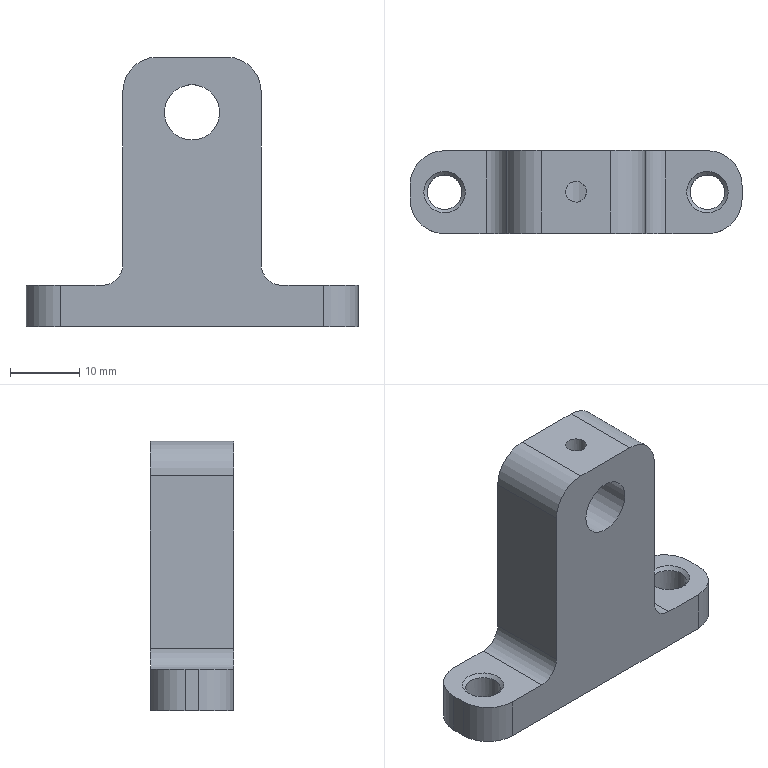Component | NX | SUPPORT_SEAT_2 | 1 solid | 24 faces | volume 10293 mm3 | cylinder 12 | plane 10 | cone 2 | commonest cylinder face diameters 10 x6 6 x2 5 x2 8 x1 3 x1